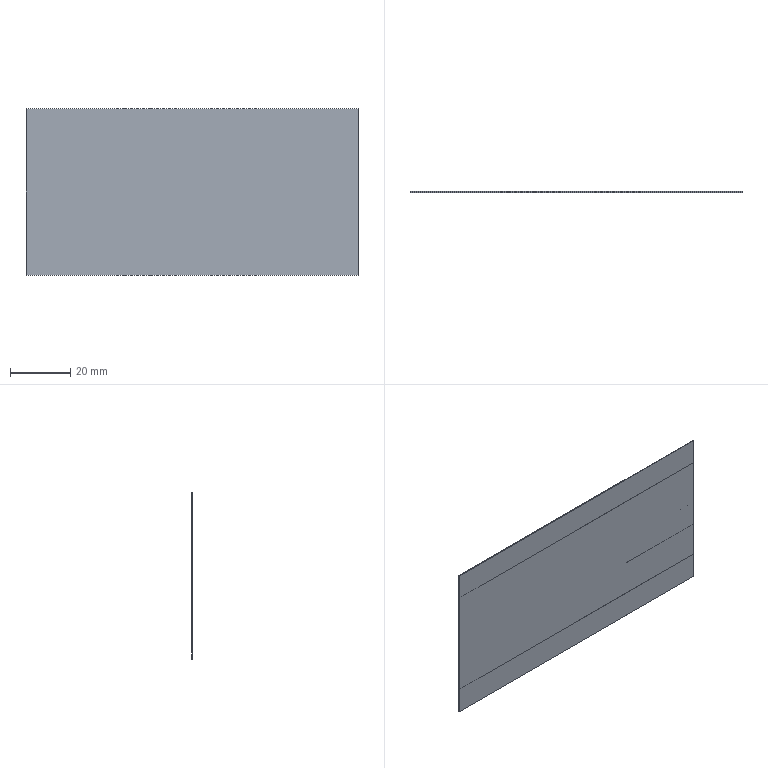Component | SolidWorks | OuterBagStorageAssembly-1_PackagingBagShort-1 | 1 solid | 16 faces | box 110.3 x 0.45 x 55.2 mm | volume 1281 mm3 | plane 16
build123d program:
from build123d import *

# Parameters (mm, degrees)
SKETCH1_W           = 55.2
SKETCH1_H           = 110.3
BOSS_EXTRUDE1_DEPTH = 0.0375
SKETCH2_W           = 9
SKETCH2_H           = 110.3
BOSS_EXTRUDE2_DEPTH = 0.15
SKETCH3_W           = 55.2
SKETCH3_H           = 110.3
BOSS_EXTRUDE3_DEPTH = 0.075
SKETCH4_W           = 9
SKETCH4_H           = 110.3
BOSS_EXTRUDE4_DEPTH = 0.15
SKETCH5_W           = 8.9
SKETCH5_H           = 0.08
CUT_EXTRUDE1_DEPTH  = 114.701


with BuildPart() as part:
    # Sketch1 → Boss-Extrude1 (new, symmetric)
    with BuildSketch(Plane(origin=(0, 0, 0), x_dir=(1, 0, 0), z_dir=(0, 1, 0))):
        Rectangle(SKETCH1_W, SKETCH1_H)
    extrude(amount=BOSS_EXTRUDE1_DEPTH, both=True)

    # Sketch2 → Boss-Extrude2 (add)
    with BuildSketch(Plane(origin=(0, 0.0375, 0), x_dir=(1, 0, 0), z_dir=(0, 1, 0))):
        with Locations((-23.1, 0)):
            Rectangle(SKETCH2_W, SKETCH2_H)
        with Locations((23.1, 0)):
            Rectangle(SKETCH2_W, SKETCH2_H)
    extrude(amount=BOSS_EXTRUDE2_DEPTH)

    # Sketch3 → Boss-Extrude3 (add)
    with BuildSketch(Plane(origin=(0, 0.1875, 0), x_dir=(1, 0, 0), z_dir=(0, 1, 0))):
        Rectangle(SKETCH3_W, SKETCH3_H)
    extrude(amount=BOSS_EXTRUDE3_DEPTH)

    # Sketch4 → Boss-Extrude4 (add)
    with BuildSketch(Plane(origin=(0, 0.2625, 0), x_dir=(1, 0, 0), z_dir=(0, 1, 0))):
        with Locations((-1.9, 0)):
            Rectangle(SKETCH4_W, SKETCH4_H)
    extrude(amount=BOSS_EXTRUDE4_DEPTH)

    # Sketch5 → Cut-Extrude1 (cut, through all)
    with BuildSketch(Plane.XY.offset(55.15)):
        with Locations((-1.85, 0.3025)):
            Rectangle(SKETCH5_W, SKETCH5_H)
    extrude(amount=-CUT_EXTRUDE1_DEPTH, mode=Mode.SUBTRACT)


solid = part.part

# Placed as in the assembly
solid = solid.moved(Location((-314.796, 200.173, 374.168), (0, -90, 0)))